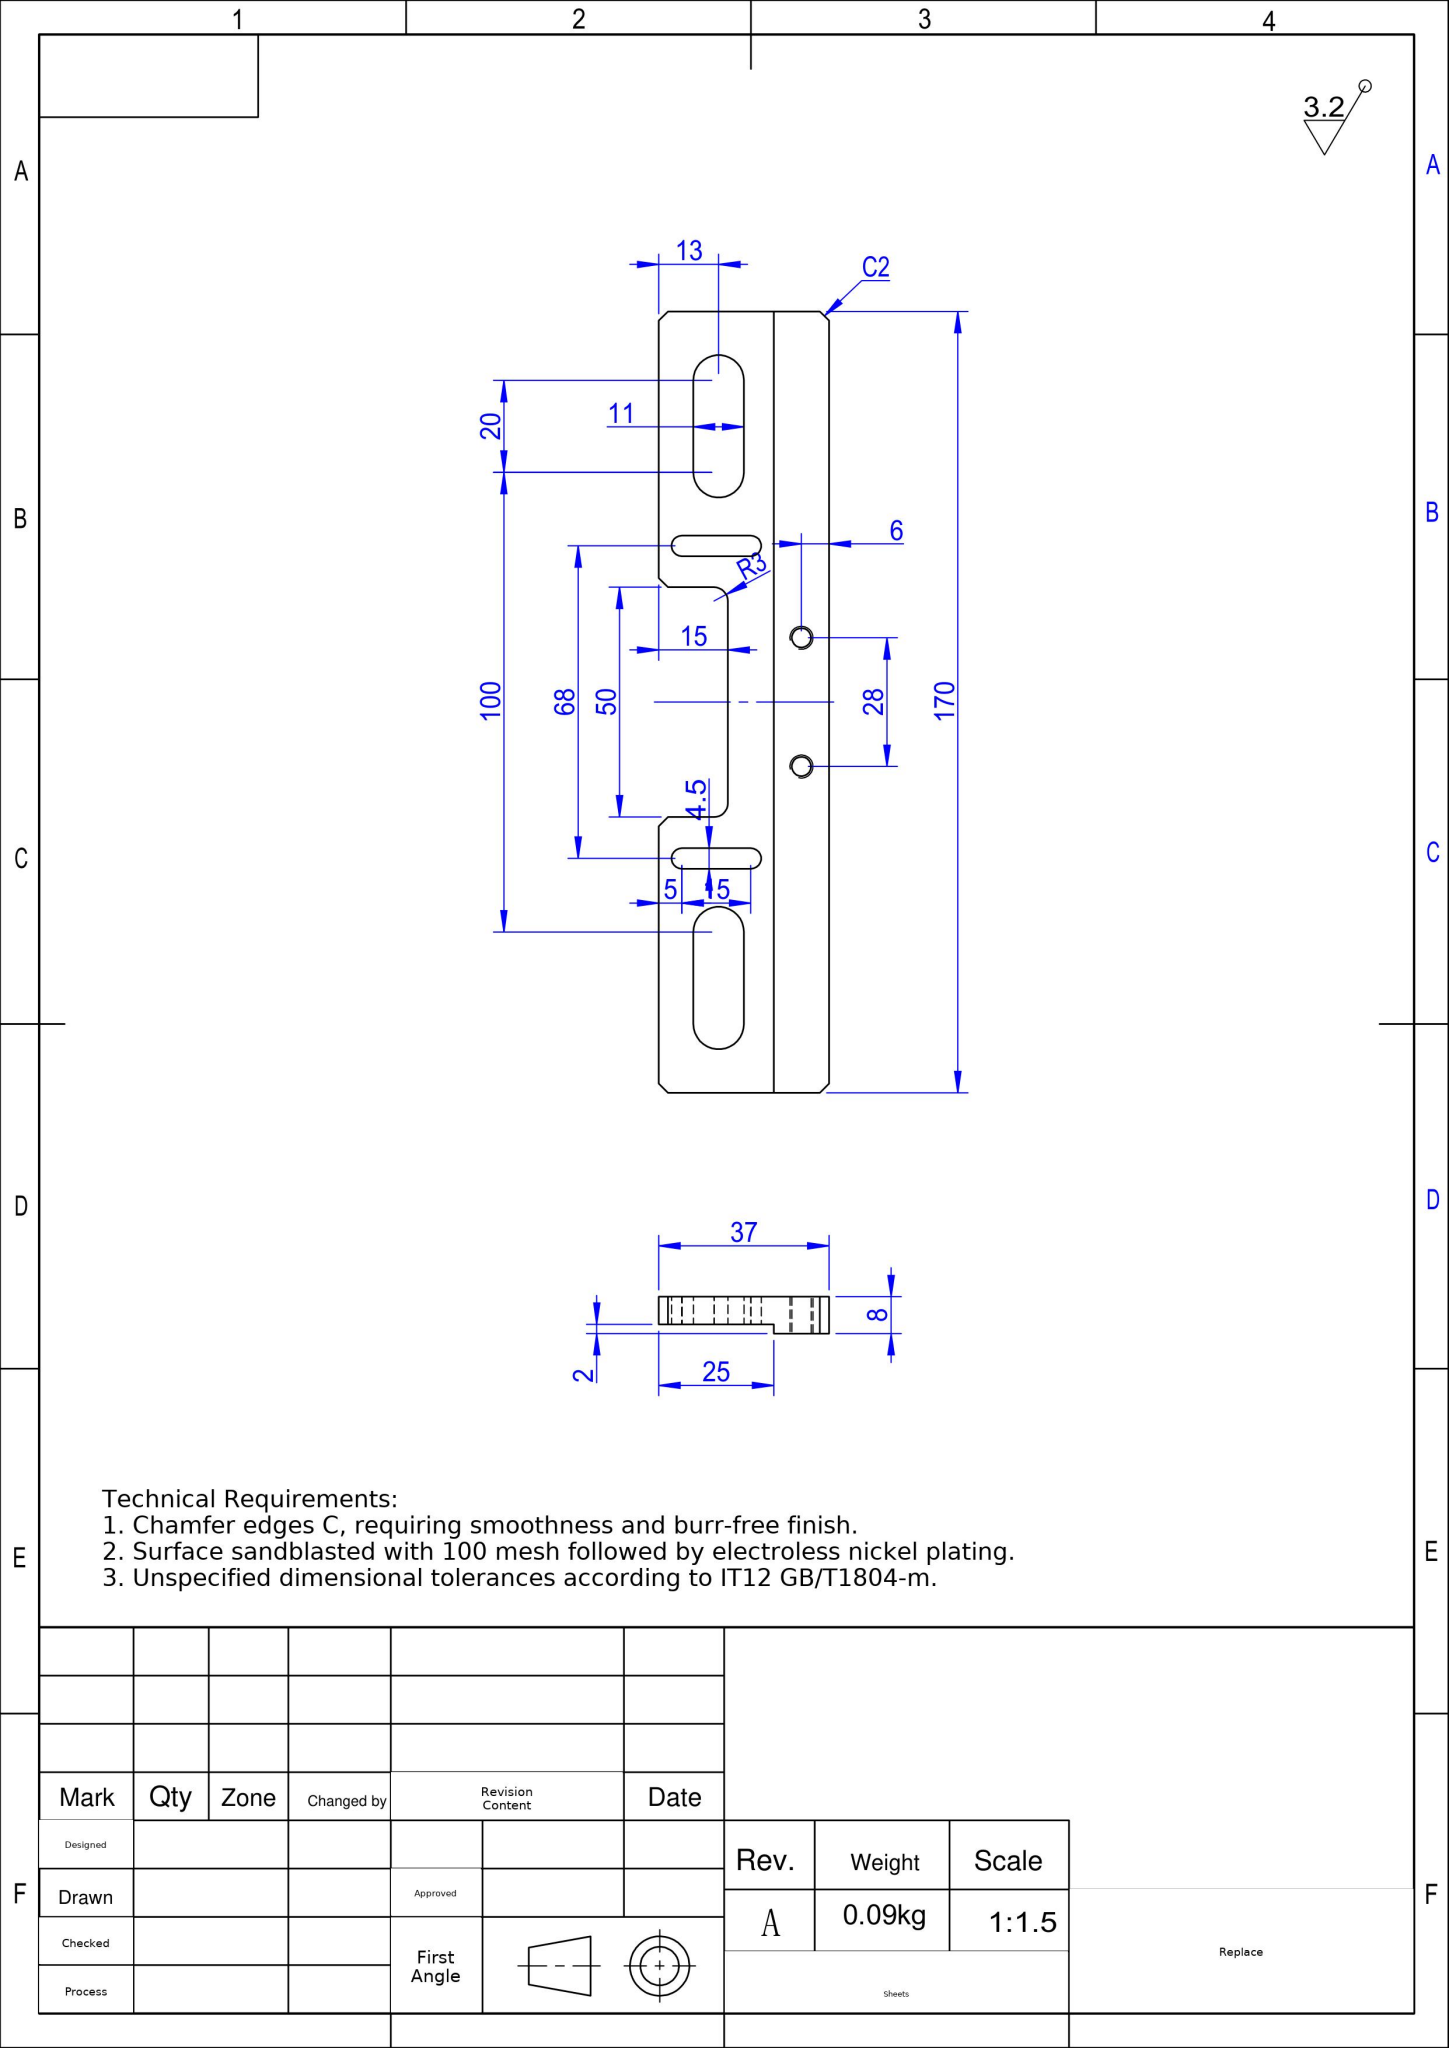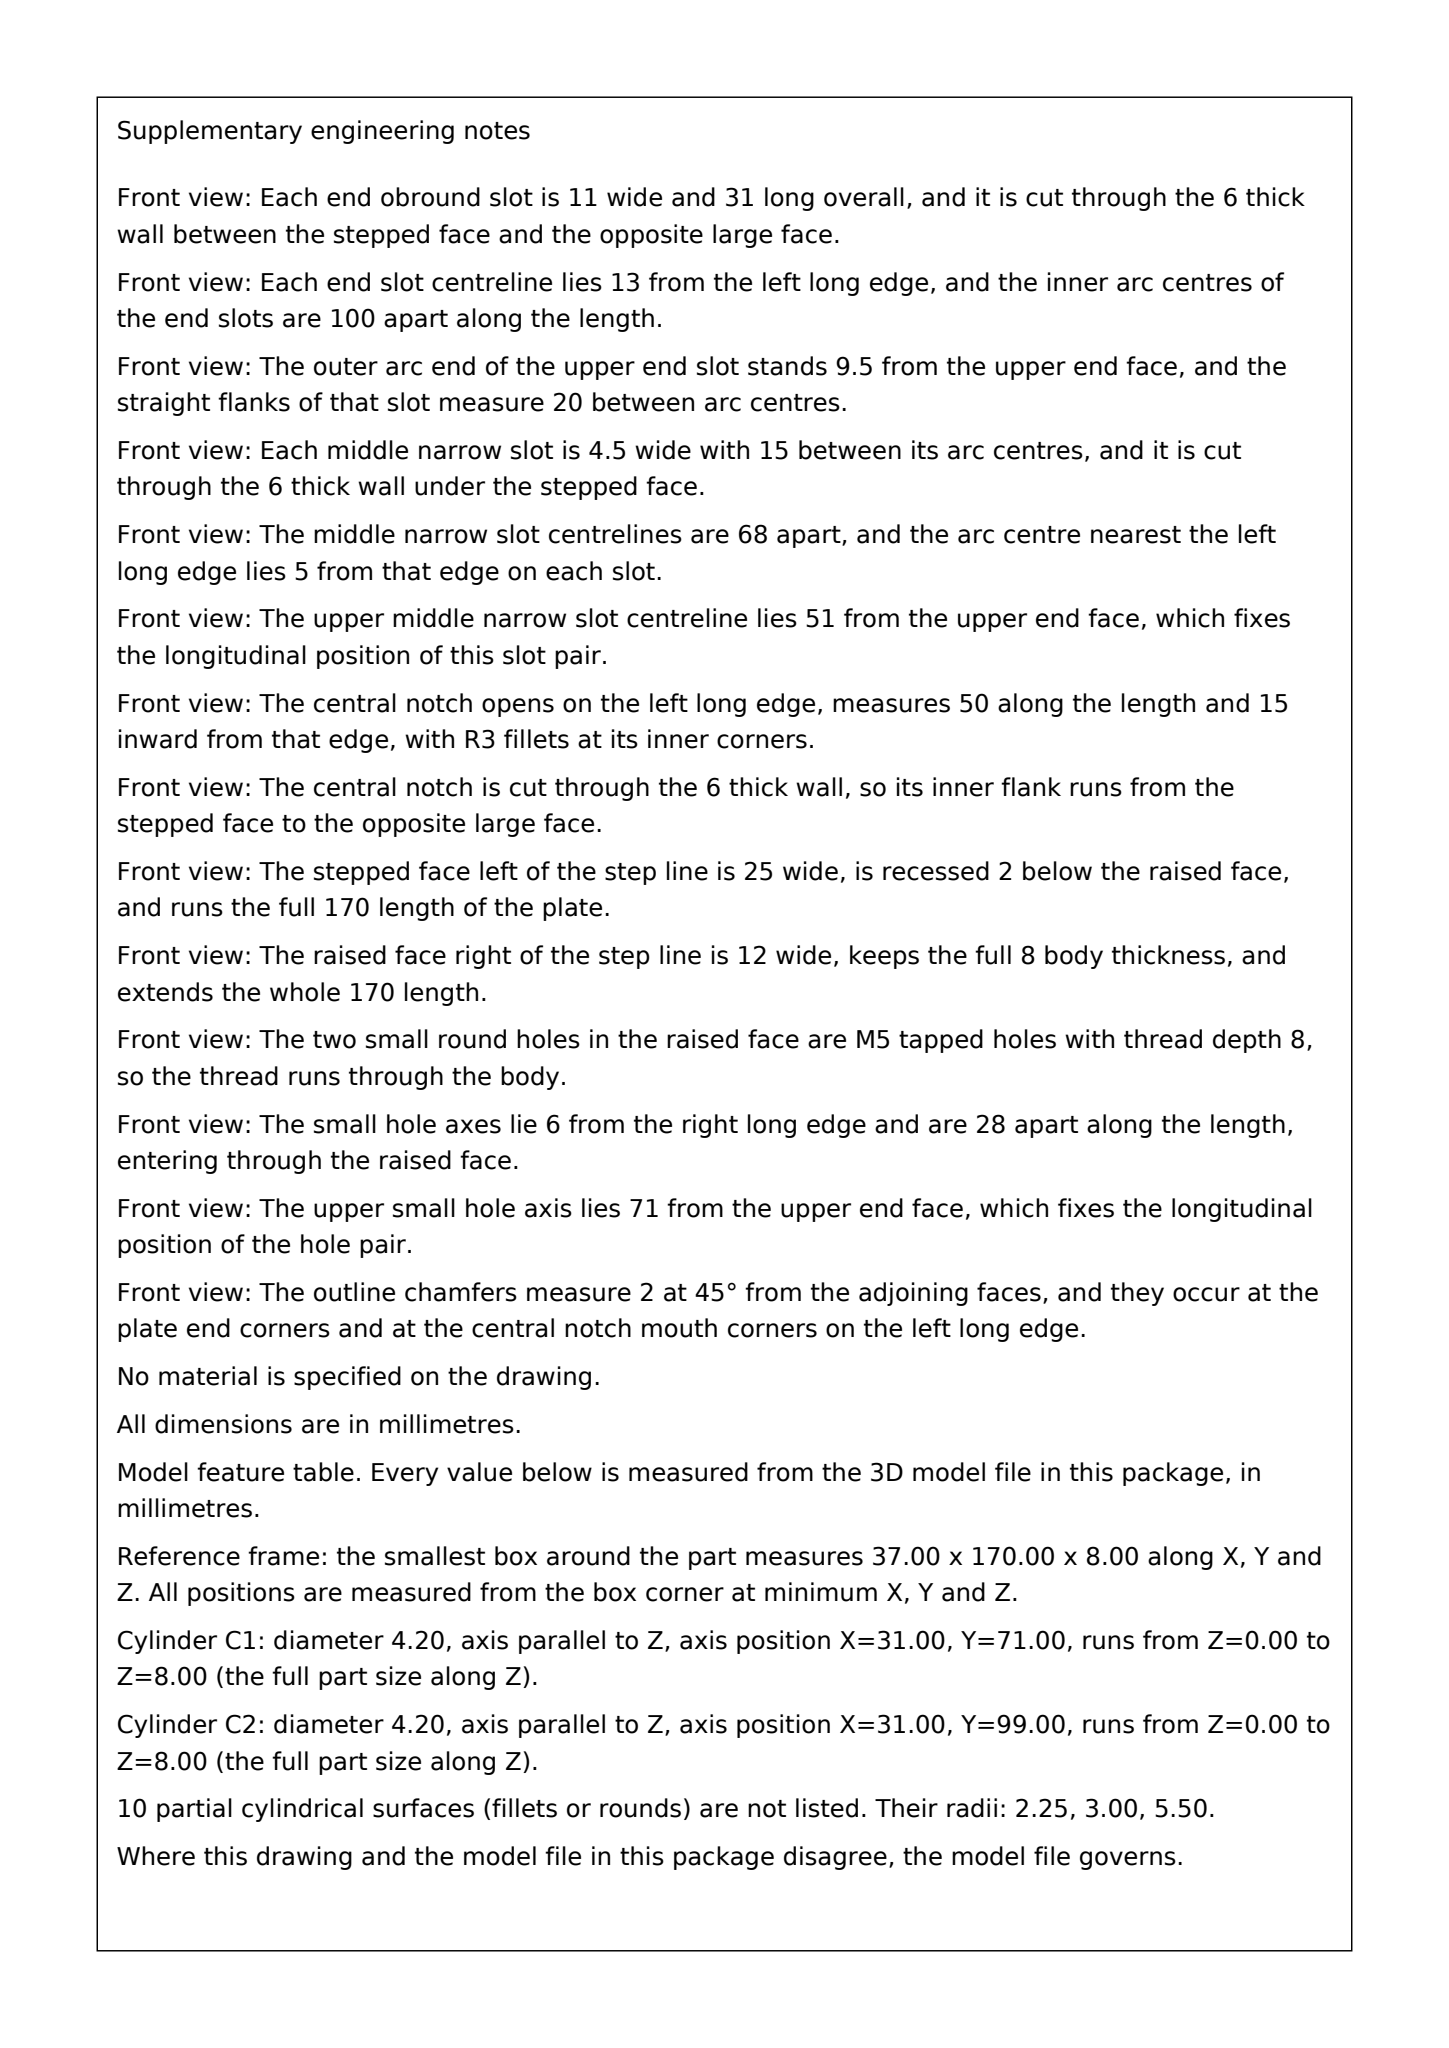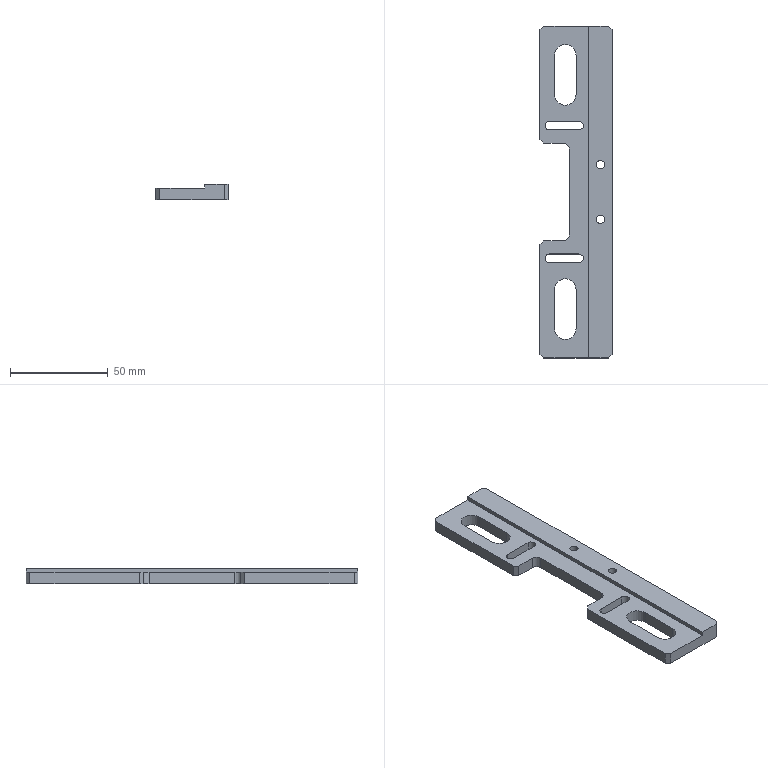Part | SolidWorks | mm | 1 solid | 42 faces | box 37 x 170 x 8 mm | volume 32260 mm3 | plane 26 | cylinder 16 | commonest cylinder face diameters 4.5 x6 4.2 x4 11 x4 6 x2
Drawing notes:
LOWER SLOT: 4.5 WIDE x 15 C-C, 5 FROM LEFT EDGE | from the solid: Ø4.5 thru-pocket cyls at (5,51) & (20,51), z-len 6; x=0 face = left edge
build123d program:
from build123d import *

# Parameters (mm, degrees)
SKETCH1_W           = 37
SKETCH1_H           = 170
BOSS_EXTRUDE1_DEPTH = 4
CHAMFER1_SIZE       = 2
CUT_EXTRUDE5_DEPTH  = 88.357
SKETCH17_W          = 25
SKETCH17_H          = 170
CUT_EXTRUDE6_DEPTH  = 2
CUT_EXTRUDE7_DEPTH  = 88.357
M5_TAPPED_HOLE1_D   = 4.2
CUT_EXTRUDE8_DEPTH  = 88.357
CHAMFER2_SIZE       = 2


with BuildPart() as part:
    # Sketch1 → Boss-Extrude1 (new, symmetric)
    with BuildSketch(Plane.XY):
        Rectangle(SKETCH1_W, SKETCH1_H)
    extrude(amount=BOSS_EXTRUDE1_DEPTH, both=True)

    # Chamfer1
    chamfer1_edges = [part.edges().sort_by_distance(p)[0] for p in [
        (-18.5, 85, 0),
        (18.5, 85, 0),
        (18.5, -85, 0),
        (-18.5, -85, 0),
    ]]
    chamfer(chamfer1_edges, length=CHAMFER1_SIZE)

    # Sketch16 → Cut-Extrude5 (cut, through all)
    with BuildSketch(Plane.XY.offset(4)):
        with BuildLine():
            Line((0, 70), (0, 50))
            ThreePointArc((0, 50), (-5.5, 44.5), (-11, 50))
            Line((-11, 50), (-11, 70))
            ThreePointArc((-11, 70), (-5.5, 75.5), (0, 70))
        make_face()
        with BuildLine():
            Line((0, -50), (0, -70))
            ThreePointArc((0, -70), (-5.5, -75.5), (-11, -70))
            Line((-11, -70), (-11, -50))
            ThreePointArc((-11, -50), (-5.5, -44.5), (0, -50))
        make_face()
    extrude(amount=-CUT_EXTRUDE5_DEPTH, mode=Mode.SUBTRACT)

    # Sketch17 → Cut-Extrude6 (cut)
    with BuildSketch(Plane.XY.offset(4)):
        with Locations((-6, 0)):
            Rectangle(SKETCH17_W, SKETCH17_H)
    extrude(amount=-CUT_EXTRUDE6_DEPTH, mode=Mode.SUBTRACT)

    # Sketch18 → Cut-Extrude7 (cut, through all)
    with BuildSketch(Plane(origin=(0, 0, -4), x_dir=(-1, 0, 0), z_dir=(0, 0, -1))):
        with BuildLine():
            Line((13.5, 31.75), (-1.5, 31.75))
            ThreePointArc((-1.5, 31.75), (-3.75, 34), (-1.5, 36.25))
            Line((-1.5, 36.25), (13.5, 36.25))
            ThreePointArc((13.5, 36.25), (15.75, 34), (13.5, 31.75))
        make_face()
    cut_extrude7 = extrude(amount=-CUT_EXTRUDE7_DEPTH, mode=Mode.SUBTRACT)

    # Mirror1: Cut-Extrude7 across plane
    add(cut_extrude7.mirror(Plane.ZX), mode=Mode.SUBTRACT)

    # M5 Tapped Hole1 (through all)
    with Locations(Plane.XY.offset(4)):
        with Locations((12.5, 14), (12.5, -14)):
            Hole(M5_TAPPED_HOLE1_D / 2)

    # Sketch21 → Cut-Extrude8 (cut, through all)
    with BuildSketch(Plane.XY.offset(4)):
        with BuildLine():
            Line((-6.5, 25), (-18.5, 25))
            Line((-18.5, 25), (-18.5, -25))
            Line((-18.5, -25), (-6.5, -25))
            ThreePointArc((-6.5, -25), (-4.379, -24.121), (-3.5, -22))
            Line((-3.5, -22), (-3.5, 22))
            ThreePointArc((-3.5, 22), (-4.379, 24.121), (-6.5, 25))
        make_face()
    extrude(amount=-CUT_EXTRUDE8_DEPTH, mode=Mode.SUBTRACT)

    # Chamfer2
    chamfer2_edges = [part.edges().sort_by_distance(p)[0] for p in [
        (-18.5, -25, -1),
        (-18.5, 25, -1),
    ]]
    chamfer(chamfer2_edges, length=CHAMFER2_SIZE)


solid = part.part